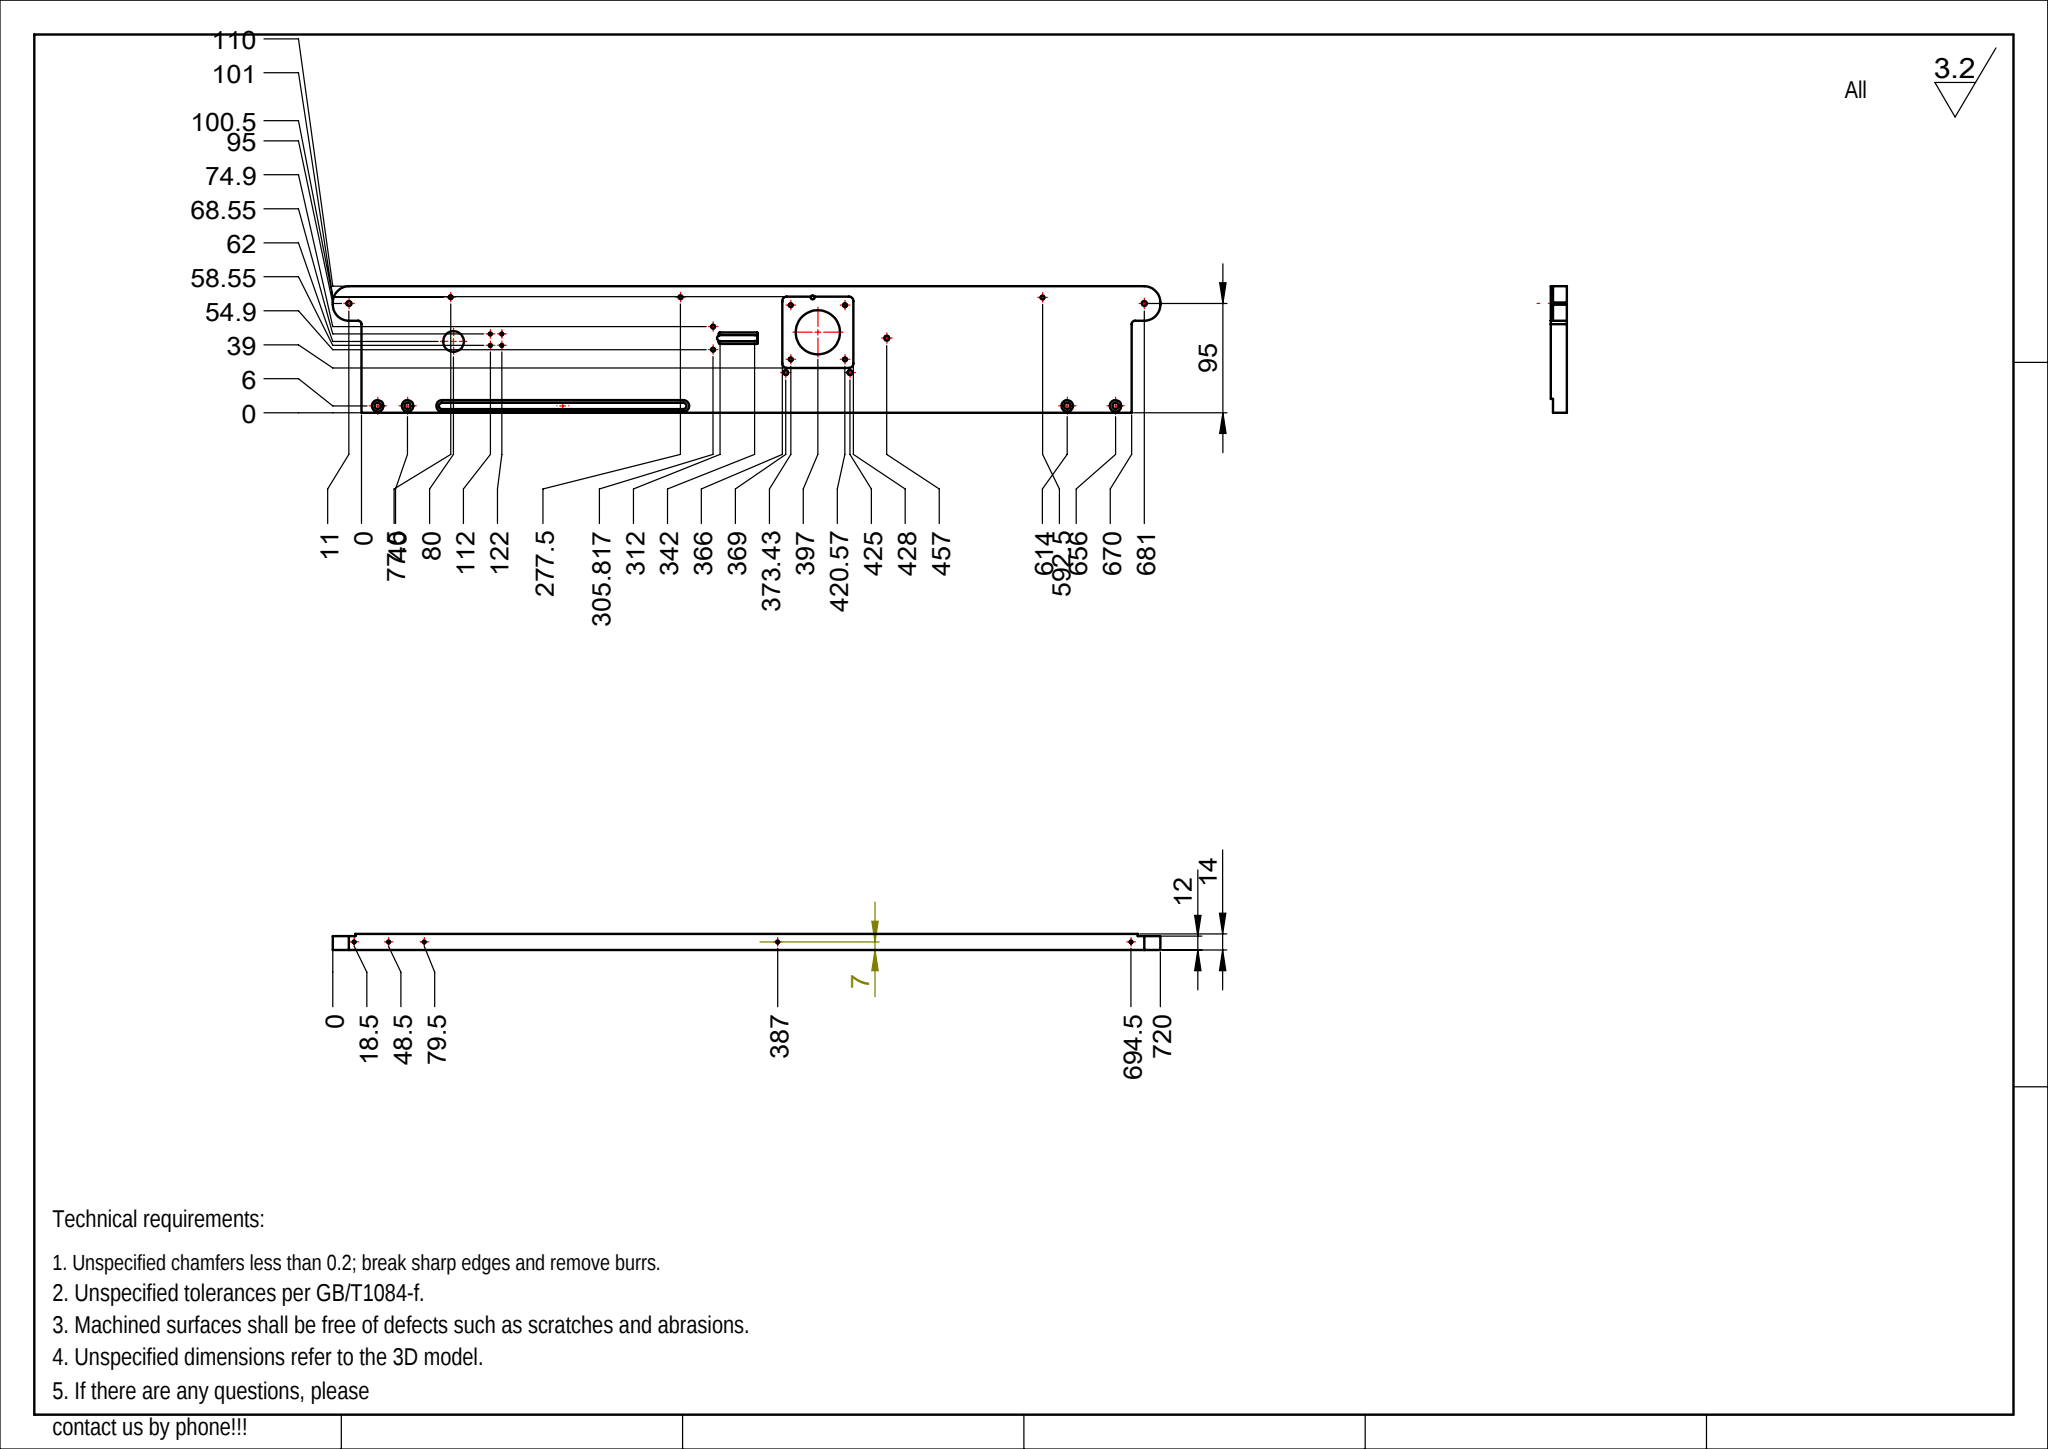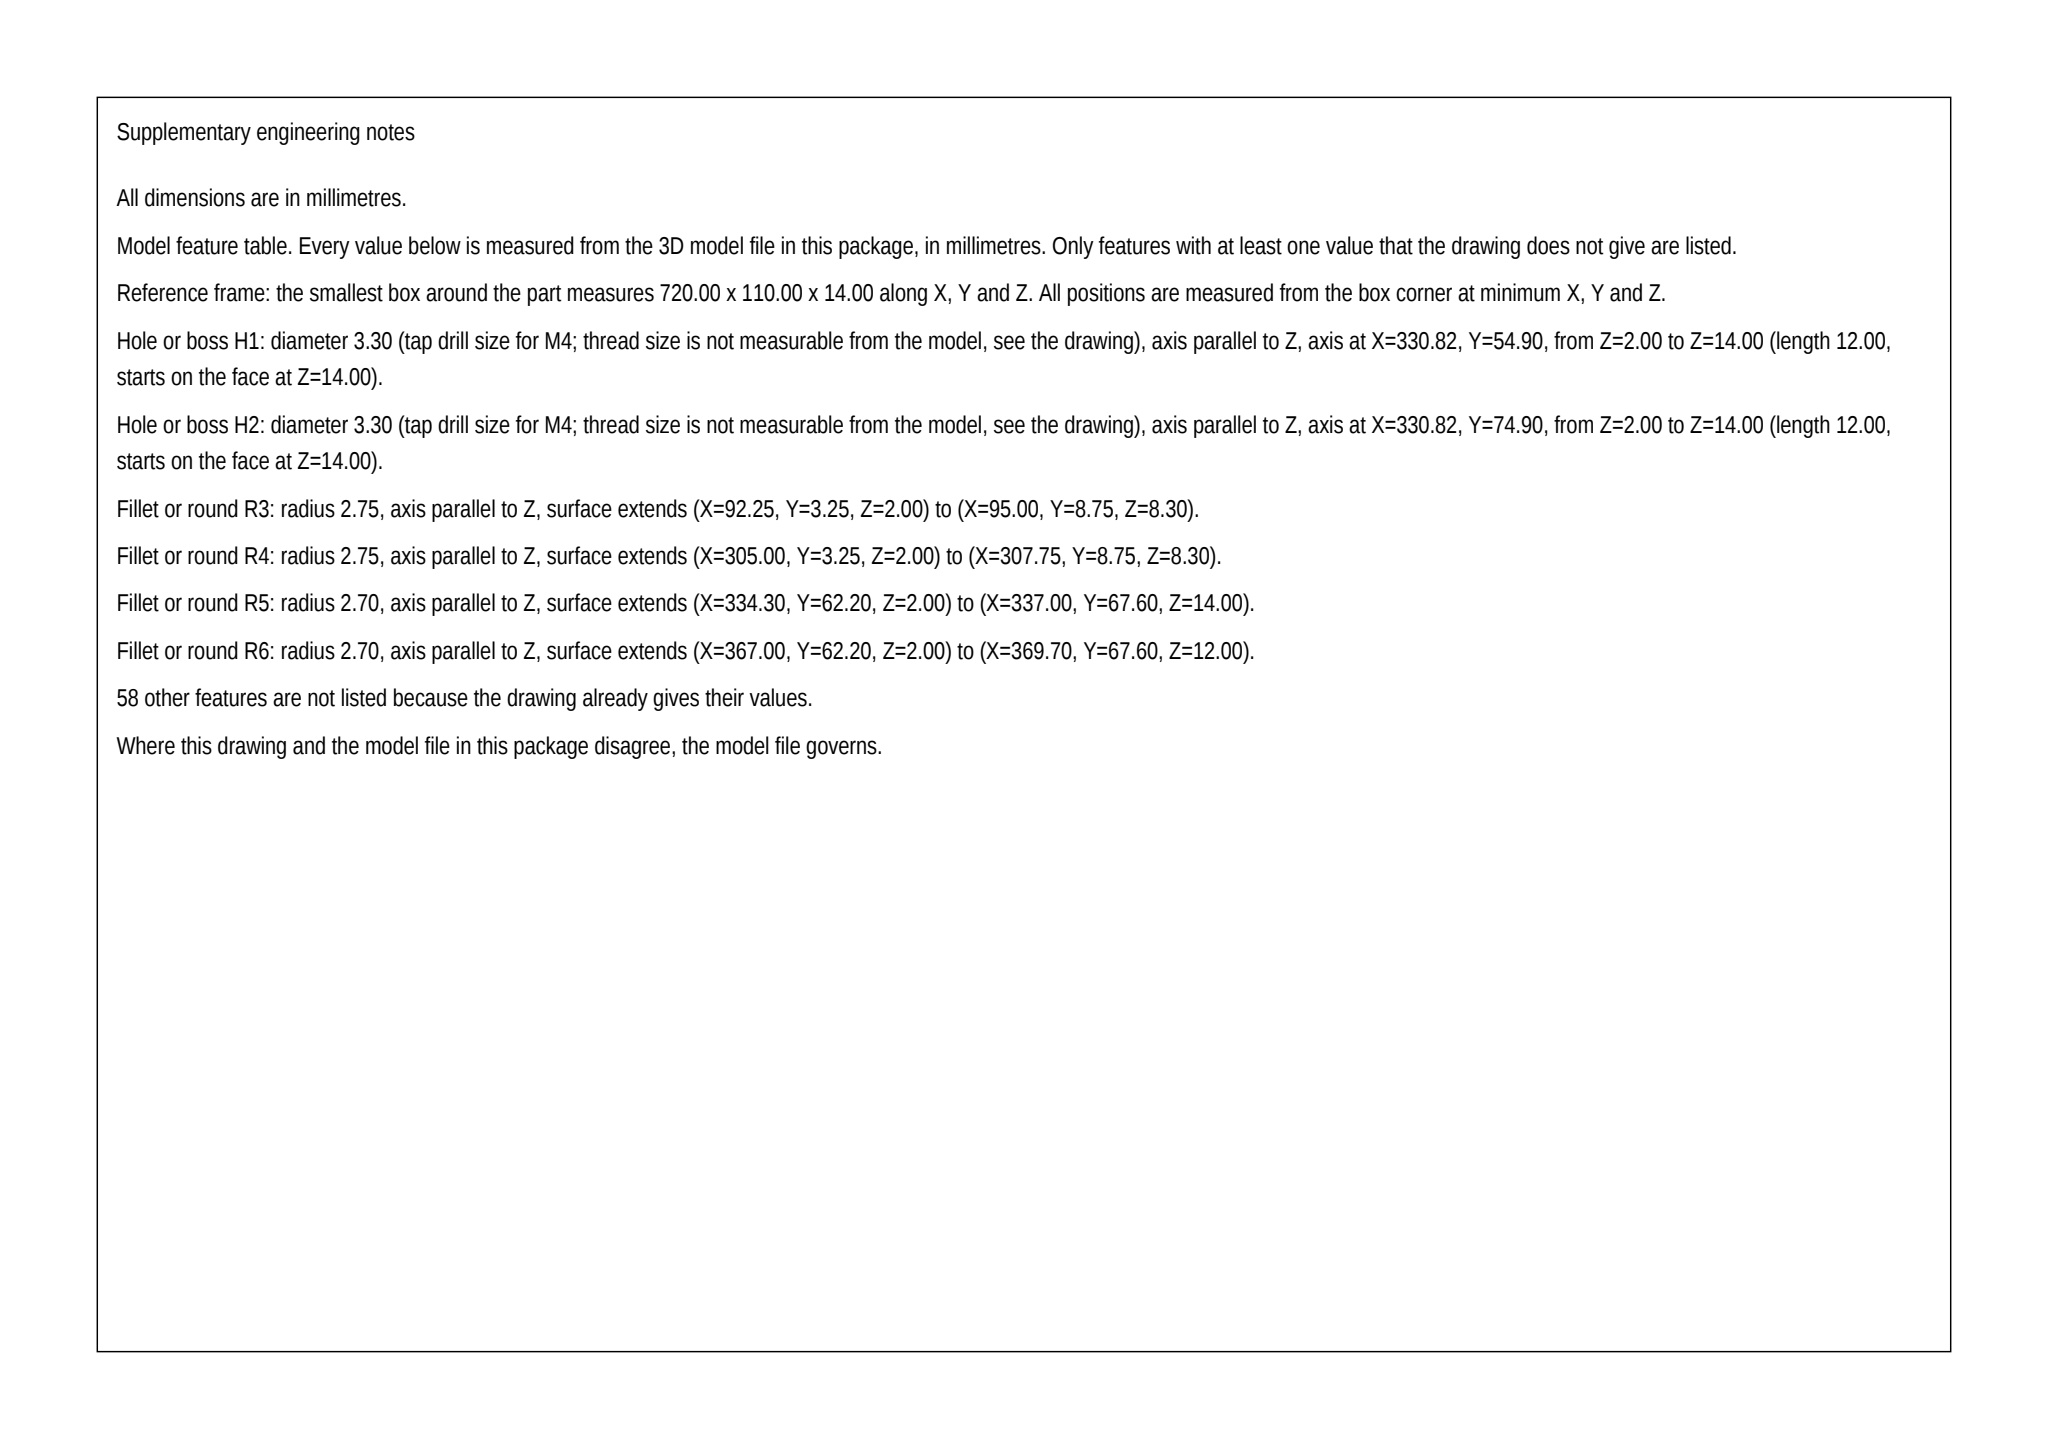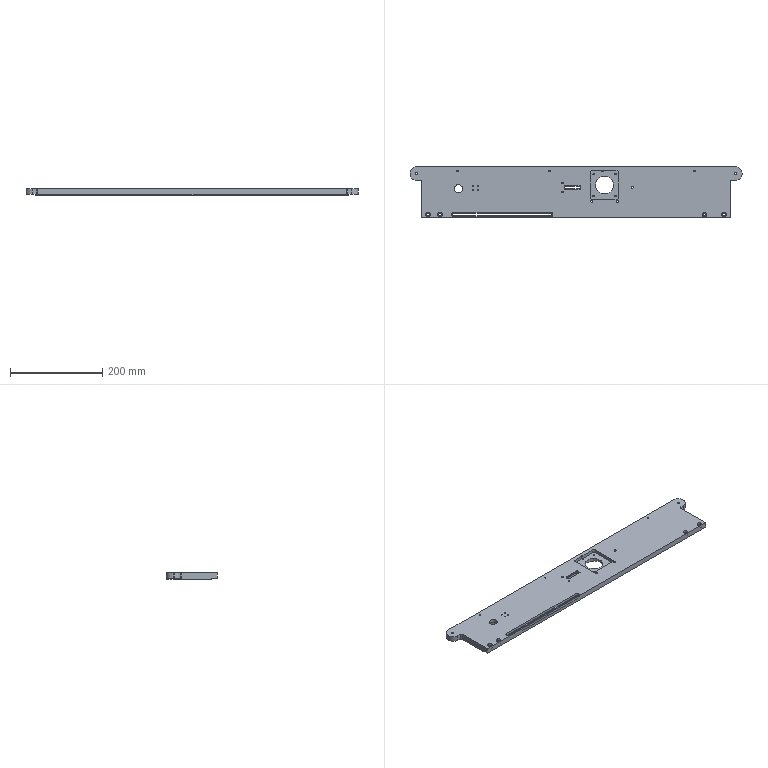Part | SolidWorks | mm | 1 solid | 167 faces | box 720 x 110 x 14 mm | volume 955366 mm3 | cylinder 109 | plane 44 | cone 14 | commonest cylinder face diameters 2.5 x22 3.3 x20 32 x12 10 x11 5.5 x11 4.2 x10 28 x4 8 x4
Drawing notes:
PLATE 720 x 110 x 14 THK | from the solid: bbox_xyz 720 x 110 x 14
STEP DP 2 TO Z12 AT BACK FACE | from the solid: z-planes 12.0 and 2.0
Ø18 THRU, CBORE Ø22 DP 7.5 AT X105 Y62 | from the solid: Ø18 z L6.5 + Ø22 z L7.5 coaxial at (105,62), sum = 14 thk
4X Ø5.5 THRU, CBORE Ø10 DP 5.7; X=39,65,639,681 AT Y6 | from the solid: Ø5.5 L6.3 + Ø10 L5.7 coaxial at (39,6),(65,6),(639,6),(681,6)
SLOT 5.5 W x 210 LG, CTRS X95-305 AT Y6, THRU; CBORE 10 W DP 5.7 | from the solid: Ø5.5/Ø10 ends at x95 & x305, y6; y-planes 3.25/8.75 and 1/11
2X Ø6 THRU 14 AT X22 & X698, Y77 | from the solid: Ø6 z L14 at (22,77) and (698,77)
4X Ø2.5 THRU 14 AT X137 & 147 x Y58.55 & 68.55 | from the solid: Ø2.5 z L14 at (137/147, 58.55/68.55)
Ø3.3 THRU 14 AT X102.5, 302.5, 417.5, 617.5 (Y100.5/100.34/100.24) | from the solid: Ø3.3 z L14 at (102.5,100.5),(302.5,100.5),(417.5,100.34),(617.5,100.24)
2X Ø3.3 DP 12 AT X330.82, Y54.9 & Y74.9 | from the solid: Ø3.3 z L12 at (330.82,54.9) and (330.82,74.9)
5X Ø4.2 DP 12: X14 & 706 AT Y95; X394 & 450 AT Y34.9; X482 AT Y64.9 | from the solid: Ø4.2 z L12 at (14,95),(394,34.9),(450,34.9),(482,64.9),(706,95)
2X OBROUND 28 W x 30 LG DP 12, CTR Y95 AT X14 & X706 | from the solid: Ø28 z L12 pairs at (14,94)&(14,96), (706,94)&(706,96)
RECESS 34 x 10 DP 2: X335.82-369.82, Y59.9-69.9 | from the solid: x-planes 335.82/369.82, y-planes 59.9/69.9, z-plane 2.0
4X Ø2 DP 2 AT X336.82 & 368.82 x Y60.9 & 68.9 | from the solid: cyl Ø2.0 z L2.0 at (336.82/368.82, 60.9/68.9)
SLOT 5.4 W x 30 LG, CTRS X337-367 AT Y64.9, DP 12 | from the solid: Ø5.4 L12 @ (337,64.9), Ø5.4 L10 @ (367,64.9); y-planes 62.2/67.6
SQ POCKET 62 x 62, CTR X422 Y70; Ø38.5 BORE DP 6.5 AT CTR | from the solid: x-planes 391/453, y-planes 39/101; Ø38.5 z L6.5 at (422,70)
4X Ø8 DP 7.5 ON 54 x 54 SQ PATTERN, CTR X422 Y70 | from the solid: Ø8 L7.5 at (395,43),(395,97),(449,43),(449,97)
4X Ø3.3 ON 47.14 SQ, CTR X422 Y70: DP 4.5 LWR, DP 6.5 UPR | from the solid: Ø3.3 L4.5 at y46.43, Ø3.3 L6.5 at y93.57, x398.43 & 445.57
7X Ø32 DP 2 FROM BACK FACE, COAX W/ Ø4.2 & Ø5.4 HOLES | from the solid: Ø32 z L2.0 at (14,95),(337,64.9),(367,64.9),(394,34.9),(450,34.9),(482,64.9),(705.85,95)
5X Ø2.5 DP 7.5, 118° PT, IN BTM EDGE AT Z7: X18.5,48.5,79.5,387,694.5 | from the solid: Ø2.5 y-axis L7.5 at x18.5,48.5,79.5,387,694.5, z7.0; cone 118°
2X Ø2.5 DP 7.5, 118° PT, IN END FACES AT Z7, Y51.5 & Y66.5 | from the solid: Ø2.5 x-axis L7.5 at (y51.5,z7) and (y66.5,z7)
BACK FACE STEP DP 2 (TO Z12) EXTENDS X25 TO X695, Y12 TO Y80 FROM BBOX MIN CORNER | from the solid: axis_planes x=25.0, x=695.0, y=12.0, y=80.0, z=12.0
NOTE 8 LOCATIONS: Ø3.3 THRU 14 AT X102.5 Y100.5; X302.5 Y100.5; X417.5 Y100.34; X617.5 Y100.24 | from the solid: cylinders dia 3.3 axis z len 14.0 at (102.5,100.5),(302.5,100.5),(417.5,100.34),(617.5,100.24)
SQ POCKET 62 x 62 BOUNDED X391 TO X453, Y39 TO Y101 (CTR X422 Y70) | from the solid: axis_planes x=391.0, x=453.0, y=39.0, y=101.0; Ø38.5 bore at (422,70)
Ø38.5 BORE AT POCKET CTR X422 Y70, DP 6.5; 4X Ø8 DP 7.5 AT X395 & X449 x Y43 & Y97 | from the solid: cylinders dia 38.5 len 6.5 at (422,70); dia 8.0 len 7.5 at (395,43),(395,97),(449,43),(449,97)
SQ POCKET 62 x 62 (X391-453, Y39-101) FLOOR AT Z7.5, i.e. DP 6.5 FROM TOP FACE (Z14); THE 4X Ø8 DP 7.5 AND 4X Ø3.3 DEPTHS ARE MEASURED FROM THIS POCKET FLOOR (Ø8 BREAKS OUT AT BACK FACE Z0) | from the solid: axis_planes z=7.5 (1) with x=391 & x=453, y=39 & y=101 pocket walls; cylinders Ø8 L7.5 at (395/449, 43/97) ending at z=0; Ø38.5 L6.5 at (422,70)
BACK-FACE STEP DP 2 (TO Z12) EXTENDS X25 TO X695 AND Y12 TO Y80 FROM THE DATUM CORNER | from the solid: axis_planes x=25, x=695, y=12, y=80 with z=12
Ø3.3 THRU 14 (NOTE 8) LOCATIONS: X102.5 & X302.5 AT Y100.5; X417.5 AT Y100.34; X617.5 AT Y100.24 | from the solid: cylinders Ø3.3 z-axis L14 at (102.5,100.5), (302.5,100.5), (417.5,100.34), (617.5,100.24)
Ø3.3 THRU 14 (NOTE 8) Y ASSIGNMENT: X102.5 & X302.5 AT Y100.5; X417.5 AT Y100.34; X617.5 AT Y100.24 (FROM PLATE MIN CORNER) | from the solid: cylinders dia 3.3 axis z len 14 at (102.5,100.5), (302.5,100.5), (417.5,100.34), (617.5,100.24)
BACK-FACE STEP DP 2 TO Z12 EXTENT: X25 TO X695, Y12 TO Y80 FROM PLATE MIN CORNER | from the solid: axis_planes x=25.0, x=695.0, y=12.0, y=80.0 with z=12.0 floor plane
X LOCATIONS FROM LEFT END (REPLACES GARBLED CALLOUTS): 2X Ø6 THRU AT X22 & X698; 4X Ø5.5 CBORE HOLES START AT X39 & X65; SLOT CTRS X95-305; Ø3.3 THRU AT X102.5 & X617.5 | from the solid: cylinders dia 6.0 at x22 & x698 y77; dia 5.5 at x39, x65, x95, x305; dia 3.3 thru at x102.5 and x617.5